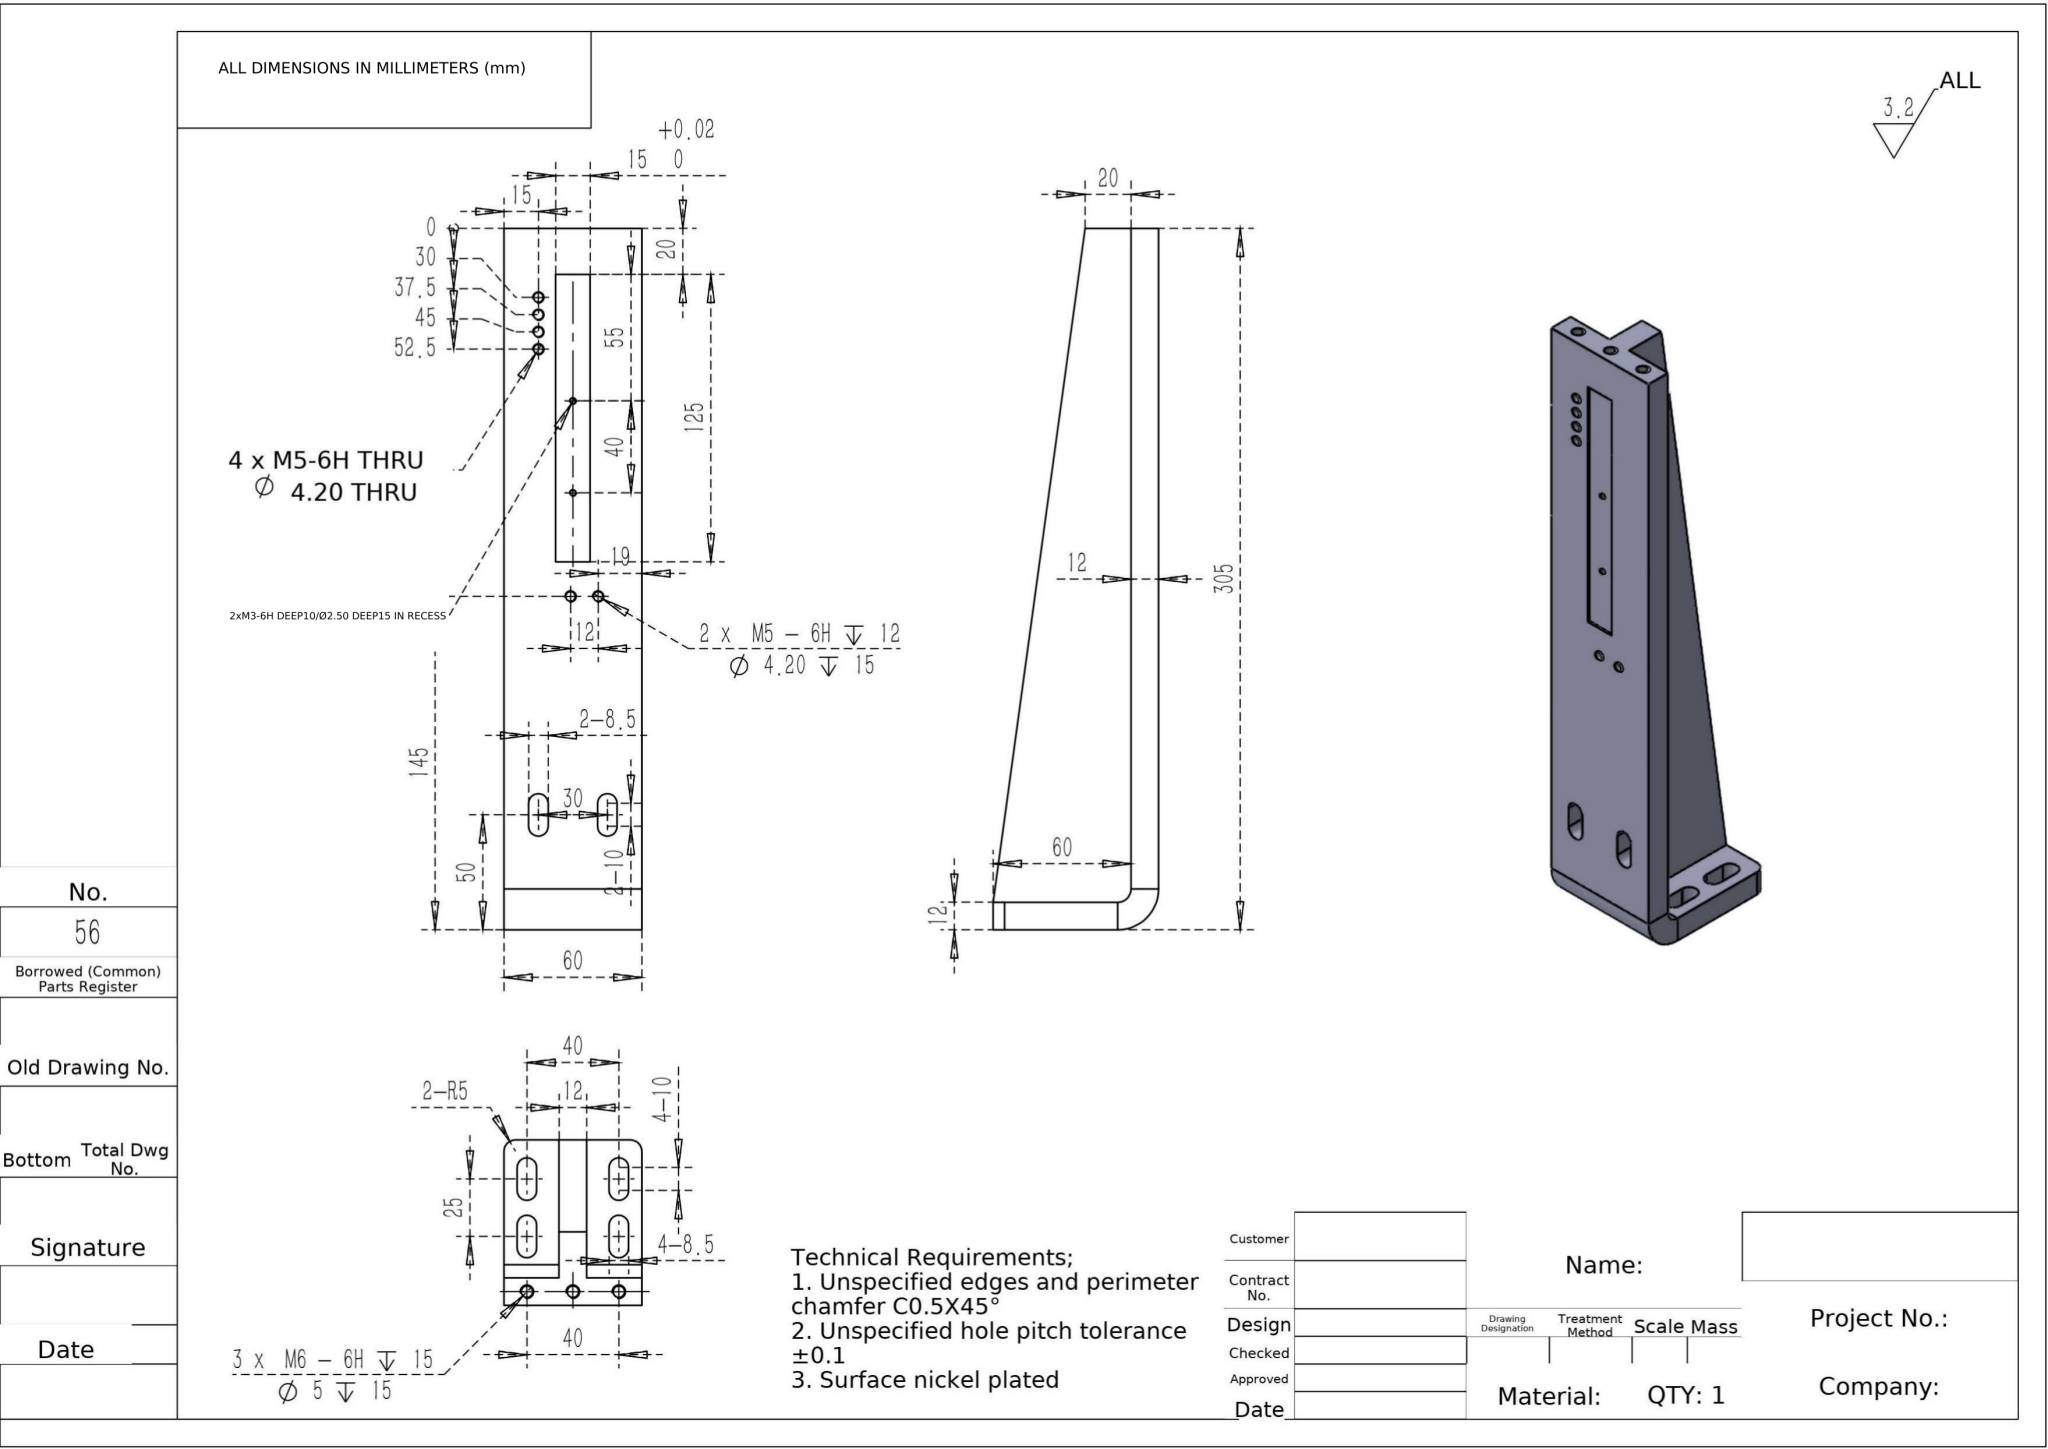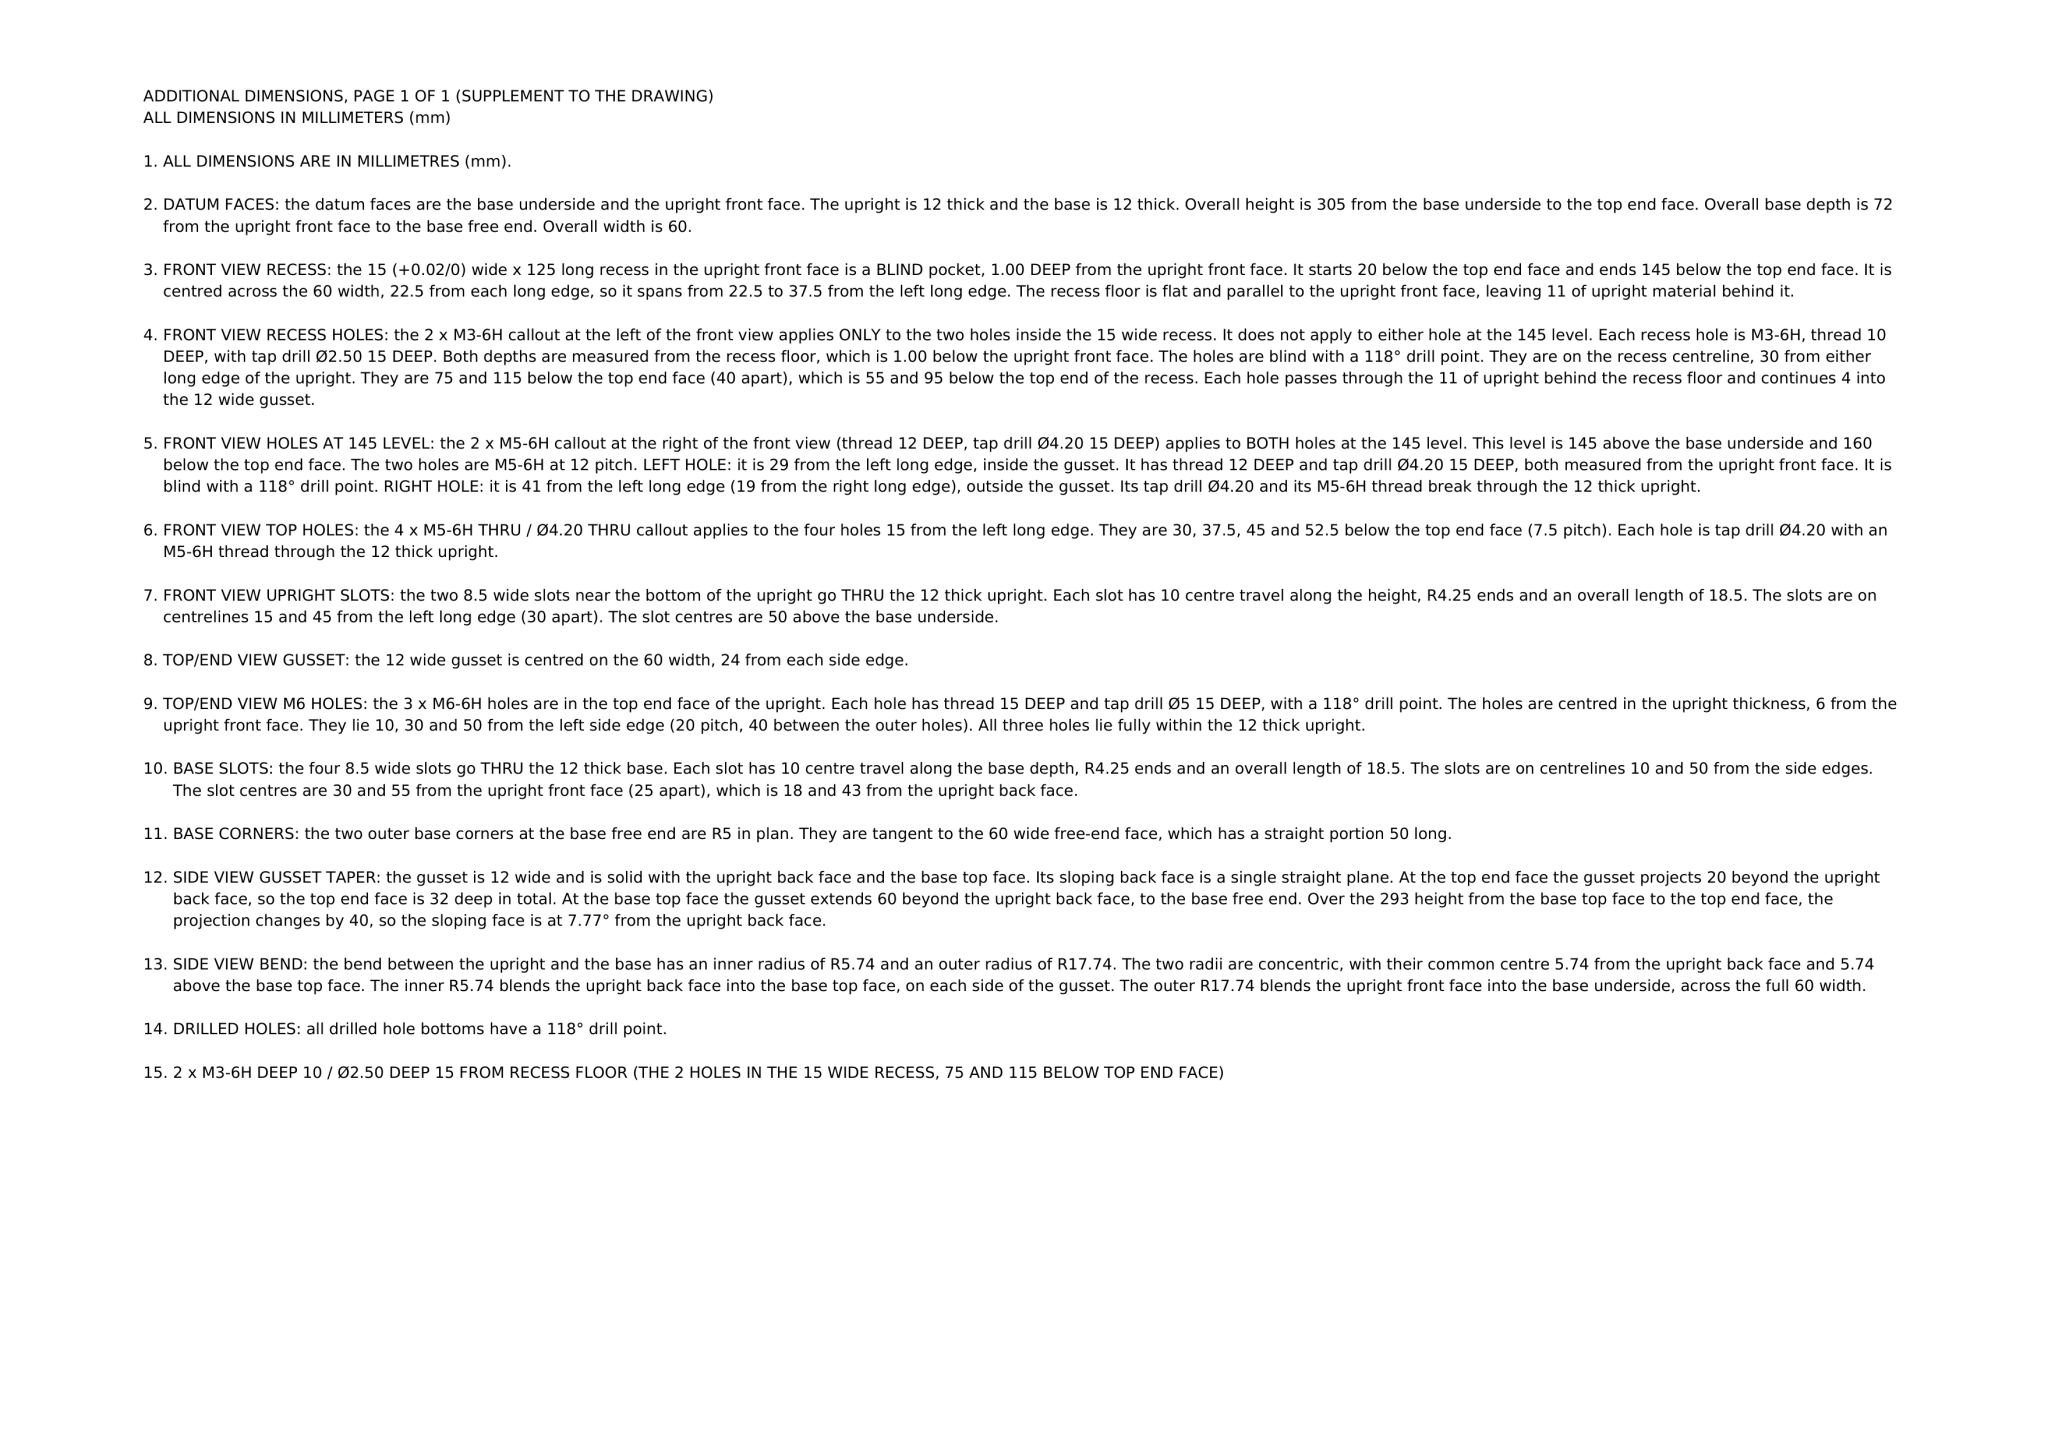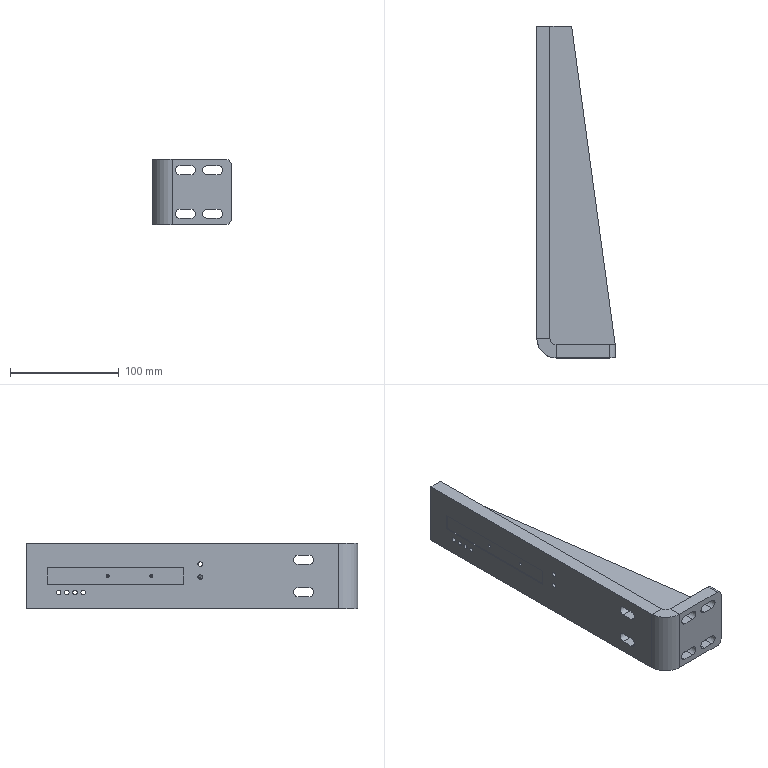Part | NX | mm | 1 solid | 85 faces | box 72 x 305 x 60 mm | volume 385411 mm3 | cylinder 39 | plane 34 | cone 12 | commonest cylinder face diameters 4.2 x12 8.5 x12 5 x6 2.5 x4 11.473 x2 10 x2 35.473 x1